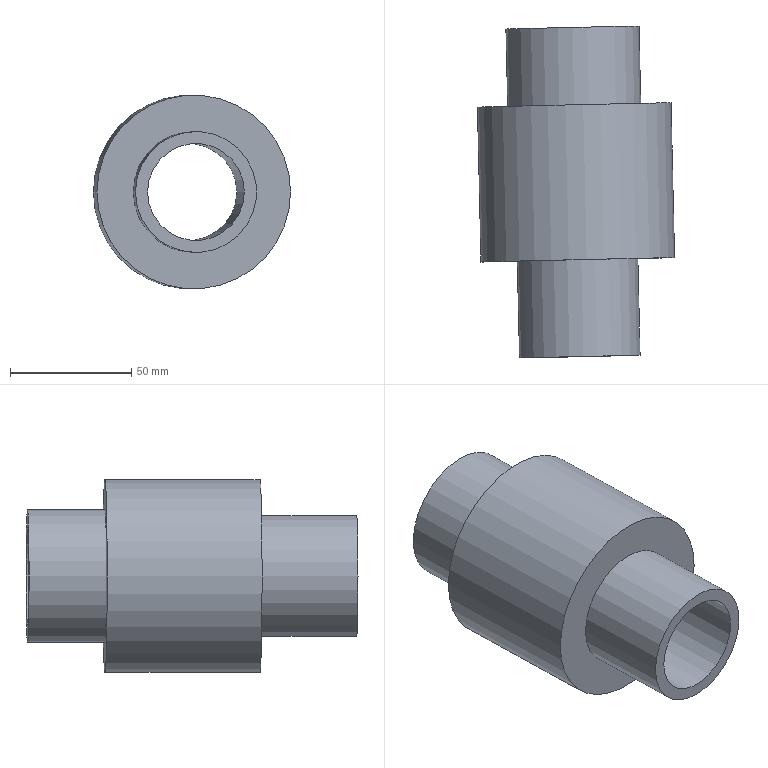Component | NX | 3 | 1 solid | 8 faces | box 81.44 x 137.16 x 80 mm | volume 305363 mm3 | plane 4 | cylinder 4 | commonest cylinder face diameters 40 x1 50 x1 80 x1 55 x1
STEP:
#1=CARTESIAN_POINT('',(0.,0.,0.));
#2=DIRECTION('',(0.,0.,1.));
#3=DIRECTION('',(1.,0.,0.));
#4=AXIS2_PLACEMENT_3D('',#1,#2,#3);
#5=CARTESIAN_POINT('',(-404.632,524.19,168.288));
#6=VERTEX_POINT('',#5);
#7=CARTESIAN_POINT('',(-384.637,524.647,168.288));
#8=DIRECTION('',(-0.02285,0.9997,0.));
#9=DIRECTION('',(-0.9997,-0.02285,0.));
#10=AXIS2_PLACEMENT_3D('',#7,#8,#9);
#11=CIRCLE('',#10,20.);
#12=CARTESIAN_POINT('',(-357.144,525.275,168.288));
#13=DIRECTION('',(0.02285,-0.9997,0.));
#14=DIRECTION('',(0.9997,0.02285,-0.));
#15=AXIS2_PLACEMENT_3D('',#12,#13,#14);
#16=PLANE('',#15);
#17=CARTESIAN_POINT('',(-47.5,-0.));
#18=CARTESIAN_POINT('',(-47.5,34.641));
#19=CARTESIAN_POINT('',(-17.5,17.321));
#20=CARTESIAN_POINT('',(12.5,-0.));
#21=CARTESIAN_POINT('',(-17.5,-17.321));
#22=CARTESIAN_POINT('',(-47.5,-34.641));
#23=CARTESIAN_POINT('',(-47.5,-0.));
#24=(BOUNDED_CURVE()B_SPLINE_CURVE(2,(#17,#18,#19,#20,#21,#22,#23),.UNSPECIFIED.,.T.,.F.)B_SPLINE_CURVE_WITH_KNOTS((1,2,2,2,2,1),(-2.094,0.,2.094,4.189,6.283,8.378),.UNSPECIFIED.)CURVE()GEOMETRIC_REPRESENTATION_ITEM()RATIONAL_B_SPLINE_CURVE((1.,0.5,1.,0.5,1.,0.5,1.))REPRESENTATION_ITEM(''));
#25=(GEOMETRIC_REPRESENTATION_CONTEXT(2)PARAMETRIC_REPRESENTATION_CONTEXT()REPRESENTATION_CONTEXT('',''));
#26=DEFINITIONAL_REPRESENTATION('',(#24),#25);
#27=PCURVE('',#16,#26);
#28=CARTESIAN_POINT('',(-381.529,388.682,168.288));
#29=DIRECTION('',(-0.02285,0.9997,0.));
#30=DIRECTION('',(-0.9997,-0.02285,0.));
#31=AXIS2_PLACEMENT_3D('',#28,#29,#30);
#32=CYLINDRICAL_SURFACE('',#31,20.);
#33=CARTESIAN_POINT('',(0.,136.));
#34=DIRECTION('',(1.,0.));
#35=VECTOR('',#34,1.);
#36=LINE('',#33,#35);
#37=(GEOMETRIC_REPRESENTATION_CONTEXT(2)PARAMETRIC_REPRESENTATION_CONTEXT()REPRESENTATION_CONTEXT('',''));
#38=DEFINITIONAL_REPRESENTATION('',(#36),#37);
#39=PCURVE('',#32,#38);
#40=SURFACE_CURVE('',#11,(#27,#39),.PCURVE_S1.);
#41=EDGE_CURVE('',#6,#6,#40,.T.);
#42=ORIENTED_EDGE('',*,*,#41,.F.);
#43=EDGE_LOOP('',(#42));
#44=FACE_BOUND('',#43,.T.);
#45=CARTESIAN_POINT('',(-412.13,524.018,168.288));
#46=VERTEX_POINT('',#45);
#47=CARTESIAN_POINT('',(-384.637,524.647,168.288));
#48=DIRECTION('',(-0.02285,0.9997,0.));
#49=DIRECTION('',(-0.9997,-0.02285,0.));
#50=AXIS2_PLACEMENT_3D('',#47,#48,#49);
#51=CIRCLE('',#50,27.5);
#52=CARTESIAN_POINT('',(-55.,-0.));
#53=CARTESIAN_POINT('',(-55.,47.631));
#54=CARTESIAN_POINT('',(-13.75,23.816));
#55=CARTESIAN_POINT('',(27.5,-0.));
#56=CARTESIAN_POINT('',(-13.75,-23.816));
#57=CARTESIAN_POINT('',(-55.,-47.631));
#58=CARTESIAN_POINT('',(-55.,-0.));
#59=(BOUNDED_CURVE()B_SPLINE_CURVE(2,(#52,#53,#54,#55,#56,#57,#58),.UNSPECIFIED.,.T.,.F.)B_SPLINE_CURVE_WITH_KNOTS((1,2,2,2,2,1),(-2.094,0.,2.094,4.189,6.283,8.378),.UNSPECIFIED.)CURVE()GEOMETRIC_REPRESENTATION_ITEM()RATIONAL_B_SPLINE_CURVE((1.,0.5,1.,0.5,1.,0.5,1.))REPRESENTATION_ITEM(''));
#60=(GEOMETRIC_REPRESENTATION_CONTEXT(2)PARAMETRIC_REPRESENTATION_CONTEXT()REPRESENTATION_CONTEXT('',''));
#61=DEFINITIONAL_REPRESENTATION('',(#59),#60);
#62=PCURVE('',#16,#61);
#63=CARTESIAN_POINT('',(-381.529,388.682,168.288));
#64=DIRECTION('',(-0.02285,0.9997,0.));
#65=DIRECTION('',(-0.9997,-0.02285,0.));
#66=AXIS2_PLACEMENT_3D('',#63,#64,#65);
#67=CYLINDRICAL_SURFACE('',#66,27.5);
#68=CARTESIAN_POINT('',(0.,136.));
#69=DIRECTION('',(1.,0.));
#70=VECTOR('',#69,1.);
#71=LINE('',#68,#70);
#72=(GEOMETRIC_REPRESENTATION_CONTEXT(2)PARAMETRIC_REPRESENTATION_CONTEXT()REPRESENTATION_CONTEXT('',''));
#73=DEFINITIONAL_REPRESENTATION('',(#71),#72);
#74=PCURVE('',#67,#73);
#75=SURFACE_CURVE('',#51,(#62,#74),.PCURVE_S1.);
#76=EDGE_CURVE('',#46,#46,#75,.T.);
#77=ORIENTED_EDGE('',*,*,#76,.T.);
#78=EDGE_LOOP('',(#77));
#79=FACE_BOUND('',#78,.T.);
#80=ADVANCED_FACE('',(#44,#79),#16,.F.);
#81=CARTESIAN_POINT('',(-401.524,388.225,168.288));
#82=VERTEX_POINT('',#81);
#83=CARTESIAN_POINT('',(-381.529,388.682,168.288));
#84=DIRECTION('',(-0.02285,0.9997,0.));
#85=DIRECTION('',(-0.9997,-0.02285,0.));
#86=AXIS2_PLACEMENT_3D('',#83,#84,#85);
#87=CIRCLE('',#86,20.);
#88=CARTESIAN_POINT('',(0.,-0.));
#89=DIRECTION('',(1.,0.));
#90=VECTOR('',#89,1.);
#91=LINE('',#88,#90);
#92=(GEOMETRIC_REPRESENTATION_CONTEXT(2)PARAMETRIC_REPRESENTATION_CONTEXT()REPRESENTATION_CONTEXT('',''));
#93=DEFINITIONAL_REPRESENTATION('',(#91),#92);
#94=PCURVE('',#32,#93);
#95=CARTESIAN_POINT('',(-361.534,389.139,168.288));
#96=DIRECTION('',(-0.02285,0.9997,0.));
#97=DIRECTION('',(-0.9997,-0.02285,0.));
#98=AXIS2_PLACEMENT_3D('',#95,#96,#97);
#99=PLANE('',#98);
#100=CARTESIAN_POINT('',(20.,-0.));
#101=DIRECTION('',(1.,-0.));
#102=AXIS2_PLACEMENT_2D('',#100,#101);
#103=CIRCLE('',#102,20.);
#104=(GEOMETRIC_REPRESENTATION_CONTEXT(2)PARAMETRIC_REPRESENTATION_CONTEXT()REPRESENTATION_CONTEXT('',''));
#105=DEFINITIONAL_REPRESENTATION('',(#103),#104);
#106=PCURVE('',#99,#105);
#107=SURFACE_CURVE('',#87,(#94,#106),.PCURVE_S1.);
#108=EDGE_CURVE('',#82,#82,#107,.T.);
#109=ORIENTED_EDGE('',*,*,#108,.T.);
#110=CARTESIAN_POINT('',(-401.524,388.225,168.288));
#111=CARTESIAN_POINT('',(-404.632,524.19,168.288));
#112=B_SPLINE_CURVE_WITH_KNOTS('',1,(#110,#111),.UNSPECIFIED.,.F.,.F.,(2,2),(-0.,136.),.PIECEWISE_BEZIER_KNOTS.);
#113=CARTESIAN_POINT('',(6.283,0.));
#114=DIRECTION('',(0.,1.));
#115=VECTOR('',#114,1.);
#116=LINE('',#113,#115);
#117=(GEOMETRIC_REPRESENTATION_CONTEXT(2)PARAMETRIC_REPRESENTATION_CONTEXT()REPRESENTATION_CONTEXT('',''));
#118=DEFINITIONAL_REPRESENTATION('',(#116),#117);
#119=PCURVE('',#32,#118);
#120=CARTESIAN_POINT('',(0.,0.));
#121=DIRECTION('',(0.,1.));
#122=VECTOR('',#121,1.);
#123=LINE('',#120,#122);
#124=(GEOMETRIC_REPRESENTATION_CONTEXT(2)PARAMETRIC_REPRESENTATION_CONTEXT()REPRESENTATION_CONTEXT('',''));
#125=DEFINITIONAL_REPRESENTATION('',(#123),#124);
#126=PCURVE('',#32,#125);
#127=SEAM_CURVE('',#112,(#119,#126),.PCURVE_S1.);
#128=EDGE_CURVE('',#82,#6,#127,.T.);
#129=ORIENTED_EDGE('',*,*,#128,.T.);
#130=ORIENTED_EDGE('',*,*,#41,.F.);
#131=ORIENTED_EDGE('',*,*,#128,.F.);
#132=EDGE_LOOP('',(#109,#129,#130,#131));
#133=FACE_BOUND('',#132,.F.);
#134=ADVANCED_FACE('',(#133),#32,.F.);
#135=CARTESIAN_POINT('',(-406.522,388.111,168.288));
#136=VERTEX_POINT('',#135);
#137=CARTESIAN_POINT('',(-381.529,388.682,168.288));
#138=DIRECTION('',(-0.02285,0.9997,0.));
#139=DIRECTION('',(-0.9997,-0.02285,0.));
#140=AXIS2_PLACEMENT_3D('',#137,#138,#139);
#141=CIRCLE('',#140,25.);
#142=CARTESIAN_POINT('',(20.,-0.));
#143=DIRECTION('',(1.,-0.));
#144=AXIS2_PLACEMENT_2D('',#142,#143);
#145=CIRCLE('',#144,25.);
#146=(GEOMETRIC_REPRESENTATION_CONTEXT(2)PARAMETRIC_REPRESENTATION_CONTEXT()REPRESENTATION_CONTEXT('',''));
#147=DEFINITIONAL_REPRESENTATION('',(#145),#146);
#148=PCURVE('',#99,#147);
#149=CARTESIAN_POINT('',(-381.529,388.682,168.288));
#150=DIRECTION('',(-0.02285,0.9997,0.));
#151=DIRECTION('',(-0.9997,-0.02285,0.));
#152=AXIS2_PLACEMENT_3D('',#149,#150,#151);
#153=CYLINDRICAL_SURFACE('',#152,25.);
#154=CARTESIAN_POINT('',(0.,0.));
#155=DIRECTION('',(1.,0.));
#156=VECTOR('',#155,1.);
#157=LINE('',#154,#156);
#158=(GEOMETRIC_REPRESENTATION_CONTEXT(2)PARAMETRIC_REPRESENTATION_CONTEXT()REPRESENTATION_CONTEXT('',''));
#159=DEFINITIONAL_REPRESENTATION('',(#157),#158);
#160=PCURVE('',#153,#159);
#161=SURFACE_CURVE('',#141,(#148,#160),.PCURVE_S1.);
#162=EDGE_CURVE('',#136,#136,#161,.T.);
#163=ORIENTED_EDGE('',*,*,#162,.F.);
#164=EDGE_LOOP('',(#163));
#165=FACE_BOUND('',#164,.T.);
#166=ORIENTED_EDGE('',*,*,#108,.T.);
#167=EDGE_LOOP('',(#166));
#168=FACE_BOUND('',#167,.T.);
#169=ADVANCED_FACE('',(#165,#168),#99,.F.);
#170=CARTESIAN_POINT('',(-407.437,428.1,168.288));
#171=VERTEX_POINT('',#170);
#172=CARTESIAN_POINT('',(-382.443,428.672,168.288));
#173=DIRECTION('',(-0.02285,0.9997,0.));
#174=DIRECTION('',(-0.9997,-0.02285,0.));
#175=AXIS2_PLACEMENT_3D('',#172,#173,#174);
#176=CIRCLE('',#175,25.);
#177=CARTESIAN_POINT('',(0.,40.));
#178=DIRECTION('',(1.,0.));
#179=VECTOR('',#178,1.);
#180=LINE('',#177,#179);
#181=(GEOMETRIC_REPRESENTATION_CONTEXT(2)PARAMETRIC_REPRESENTATION_CONTEXT()REPRESENTATION_CONTEXT('',''));
#182=DEFINITIONAL_REPRESENTATION('',(#180),#181);
#183=PCURVE('',#153,#182);
#184=CARTESIAN_POINT('',(-357.45,429.243,168.288));
#185=DIRECTION('',(-0.02285,0.9997,0.));
#186=DIRECTION('',(-0.9997,-0.02285,0.));
#187=AXIS2_PLACEMENT_3D('',#184,#185,#186);
#188=PLANE('',#187);
#189=CARTESIAN_POINT('',(25.,-0.));
#190=DIRECTION('',(1.,-0.));
#191=AXIS2_PLACEMENT_2D('',#189,#190);
#192=CIRCLE('',#191,25.);
#193=(GEOMETRIC_REPRESENTATION_CONTEXT(2)PARAMETRIC_REPRESENTATION_CONTEXT()REPRESENTATION_CONTEXT('',''));
#194=DEFINITIONAL_REPRESENTATION('',(#192),#193);
#195=PCURVE('',#188,#194);
#196=SURFACE_CURVE('',#176,(#183,#195),.PCURVE_S1.);
#197=EDGE_CURVE('',#171,#171,#196,.T.);
#198=ORIENTED_EDGE('',*,*,#197,.F.);
#199=CARTESIAN_POINT('',(-406.522,388.111,168.288));
#200=CARTESIAN_POINT('',(-407.437,428.1,168.288));
#201=B_SPLINE_CURVE_WITH_KNOTS('',1,(#199,#200),.UNSPECIFIED.,.F.,.F.,(2,2),(0.,40.),.PIECEWISE_BEZIER_KNOTS.);
#202=CARTESIAN_POINT('',(0.,0.));
#203=DIRECTION('',(0.,1.));
#204=VECTOR('',#203,1.);
#205=LINE('',#202,#204);
#206=(GEOMETRIC_REPRESENTATION_CONTEXT(2)PARAMETRIC_REPRESENTATION_CONTEXT()REPRESENTATION_CONTEXT('',''));
#207=DEFINITIONAL_REPRESENTATION('',(#205),#206);
#208=PCURVE('',#153,#207);
#209=CARTESIAN_POINT('',(6.283,0.));
#210=DIRECTION('',(0.,1.));
#211=VECTOR('',#210,1.);
#212=LINE('',#209,#211);
#213=(GEOMETRIC_REPRESENTATION_CONTEXT(2)PARAMETRIC_REPRESENTATION_CONTEXT()REPRESENTATION_CONTEXT('',''));
#214=DEFINITIONAL_REPRESENTATION('',(#212),#213);
#215=PCURVE('',#153,#214);
#216=SEAM_CURVE('',#201,(#208,#215),.PCURVE_S1.);
#217=EDGE_CURVE('',#136,#171,#216,.T.);
#218=ORIENTED_EDGE('',*,*,#217,.F.);
#219=ORIENTED_EDGE('',*,*,#162,.T.);
#220=ORIENTED_EDGE('',*,*,#217,.T.);
#221=EDGE_LOOP('',(#198,#218,#219,#220));
#222=FACE_BOUND('',#221,.T.);
#223=ADVANCED_FACE('',(#222),#153,.T.);
#224=CARTESIAN_POINT('',(-422.433,427.758,168.288));
#225=VERTEX_POINT('',#224);
#226=CARTESIAN_POINT('',(-382.443,428.672,168.288));
#227=DIRECTION('',(-0.02285,0.9997,-0.));
#228=DIRECTION('',(-0.9997,-0.02285,0.));
#229=AXIS2_PLACEMENT_3D('',#226,#227,#228);
#230=CIRCLE('',#229,40.);
#231=CARTESIAN_POINT('',(25.,-0.));
#232=DIRECTION('',(1.,0.));
#233=AXIS2_PLACEMENT_2D('',#231,#232);
#234=CIRCLE('',#233,40.);
#235=(GEOMETRIC_REPRESENTATION_CONTEXT(2)PARAMETRIC_REPRESENTATION_CONTEXT()REPRESENTATION_CONTEXT('',''));
#236=DEFINITIONAL_REPRESENTATION('',(#234),#235);
#237=PCURVE('',#188,#236);
#238=CARTESIAN_POINT('',(-381.529,388.682,168.288));
#239=DIRECTION('',(-0.02285,0.9997,0.));
#240=DIRECTION('',(-0.9997,-0.02285,0.));
#241=AXIS2_PLACEMENT_3D('',#238,#239,#240);
#242=CYLINDRICAL_SURFACE('',#241,40.);
#243=CARTESIAN_POINT('',(0.,40.));
#244=DIRECTION('',(1.,0.));
#245=VECTOR('',#244,1.);
#246=LINE('',#243,#245);
#247=(GEOMETRIC_REPRESENTATION_CONTEXT(2)PARAMETRIC_REPRESENTATION_CONTEXT()REPRESENTATION_CONTEXT('',''));
#248=DEFINITIONAL_REPRESENTATION('',(#246),#247);
#249=PCURVE('',#242,#248);
#250=SURFACE_CURVE('',#230,(#237,#249),.PCURVE_S1.);
#251=EDGE_CURVE('',#225,#225,#250,.T.);
#252=ORIENTED_EDGE('',*,*,#251,.F.);
#253=EDGE_LOOP('',(#252));
#254=FACE_BOUND('',#253,.T.);
#255=ORIENTED_EDGE('',*,*,#197,.T.);
#256=EDGE_LOOP('',(#255));
#257=FACE_BOUND('',#256,.T.);
#258=ADVANCED_FACE('',(#254,#257),#188,.F.);
#259=CARTESIAN_POINT('',(-423.895,491.741,168.288));
#260=VERTEX_POINT('',#259);
#261=CARTESIAN_POINT('',(-343.916,493.569,168.288));
#262=VERTEX_POINT('',#261);
#263=CARTESIAN_POINT('',(-383.906,492.655,168.288));
#264=DIRECTION('',(-0.02285,0.9997,-0.));
#265=DIRECTION('',(0.9997,0.02285,-0.));
#266=AXIS2_PLACEMENT_3D('',#263,#264,#265);
#267=CIRCLE('',#266,40.);
#268=CARTESIAN_POINT('',(-3.142,104.));
#269=DIRECTION('',(1.,0.));
#270=VECTOR('',#269,1.);
#271=LINE('',#268,#270);
#272=(GEOMETRIC_REPRESENTATION_CONTEXT(2)PARAMETRIC_REPRESENTATION_CONTEXT()REPRESENTATION_CONTEXT('',''));
#273=DEFINITIONAL_REPRESENTATION('',(#271),#272);
#274=PCURVE('',#242,#273);
#275=CARTESIAN_POINT('',(-343.466,493.58,168.288));
#276=DIRECTION('',(0.02285,-0.9997,0.));
#277=DIRECTION('',(0.9997,0.02285,-0.));
#278=AXIS2_PLACEMENT_3D('',#275,#276,#277);
#279=PLANE('',#278);
#280=CARTESIAN_POINT('',(-0.4505,0.));
#281=CARTESIAN_POINT('',(-0.4505,-69.282));
#282=CARTESIAN_POINT('',(-60.451,-34.641));
#283=CARTESIAN_POINT('',(-120.451,0.));
#284=CARTESIAN_POINT('',(-60.451,34.641));
#285=CARTESIAN_POINT('',(-0.4505,69.282));
#286=CARTESIAN_POINT('',(-0.4505,0.));
#287=(BOUNDED_CURVE()B_SPLINE_CURVE(2,(#280,#281,#282,#283,#284,#285,#286),.UNSPECIFIED.,.T.,.F.)B_SPLINE_CURVE_WITH_KNOTS((1,2,2,2,2,1),(-2.094,0.,2.094,4.189,6.283,8.378),.UNSPECIFIED.)CURVE()GEOMETRIC_REPRESENTATION_ITEM()RATIONAL_B_SPLINE_CURVE((1.,0.5,1.,0.5,1.,0.5,1.))REPRESENTATION_ITEM(''));
#288=(GEOMETRIC_REPRESENTATION_CONTEXT(2)PARAMETRIC_REPRESENTATION_CONTEXT()REPRESENTATION_CONTEXT('',''));
#289=DEFINITIONAL_REPRESENTATION('',(#287),#288);
#290=PCURVE('',#279,#289);
#291=SURFACE_CURVE('',#267,(#274,#290),.PCURVE_S1.);
#292=EDGE_CURVE('',#260,#262,#291,.T.);
#293=ORIENTED_EDGE('',*,*,#292,.F.);
#294=CARTESIAN_POINT('',(-422.433,427.758,168.288));
#295=CARTESIAN_POINT('',(-423.895,491.741,168.288));
#296=B_SPLINE_CURVE_WITH_KNOTS('',1,(#294,#295),.UNSPECIFIED.,.F.,.F.,(2,2),(40.,104.),.PIECEWISE_BEZIER_KNOTS.);
#297=CARTESIAN_POINT('',(0.,0.));
#298=DIRECTION('',(0.,1.));
#299=VECTOR('',#298,1.);
#300=LINE('',#297,#299);
#301=(GEOMETRIC_REPRESENTATION_CONTEXT(2)PARAMETRIC_REPRESENTATION_CONTEXT()REPRESENTATION_CONTEXT('',''));
#302=DEFINITIONAL_REPRESENTATION('',(#300),#301);
#303=PCURVE('',#242,#302);
#304=CARTESIAN_POINT('',(6.283,0.));
#305=DIRECTION('',(0.,1.));
#306=VECTOR('',#305,1.);
#307=LINE('',#304,#306);
#308=(GEOMETRIC_REPRESENTATION_CONTEXT(2)PARAMETRIC_REPRESENTATION_CONTEXT()REPRESENTATION_CONTEXT('',''));
#309=DEFINITIONAL_REPRESENTATION('',(#307),#308);
#310=PCURVE('',#242,#309);
#311=SEAM_CURVE('',#296,(#303,#310),.PCURVE_S1.);
#312=EDGE_CURVE('',#225,#260,#311,.T.);
#313=ORIENTED_EDGE('',*,*,#312,.F.);
#314=ORIENTED_EDGE('',*,*,#251,.T.);
#315=ORIENTED_EDGE('',*,*,#312,.T.);
#316=CARTESIAN_POINT('',(-383.906,492.655,168.288));
#317=DIRECTION('',(-0.02285,0.9997,-0.));
#318=DIRECTION('',(0.9997,0.02285,-0.));
#319=AXIS2_PLACEMENT_3D('',#316,#317,#318);
#320=CIRCLE('',#319,40.);
#321=CARTESIAN_POINT('',(3.142,104.));
#322=DIRECTION('',(1.,0.));
#323=VECTOR('',#322,1.);
#324=LINE('',#321,#323);
#325=(GEOMETRIC_REPRESENTATION_CONTEXT(2)PARAMETRIC_REPRESENTATION_CONTEXT()REPRESENTATION_CONTEXT('',''));
#326=DEFINITIONAL_REPRESENTATION('',(#324),#325);
#327=PCURVE('',#242,#326);
#328=CARTESIAN_POINT('',(-0.4505,0.));
#329=CARTESIAN_POINT('',(-0.4505,-69.282));
#330=CARTESIAN_POINT('',(-60.451,-34.641));
#331=CARTESIAN_POINT('',(-120.451,0.));
#332=CARTESIAN_POINT('',(-60.451,34.641));
#333=CARTESIAN_POINT('',(-0.4505,69.282));
#334=CARTESIAN_POINT('',(-0.4505,0.));
#335=(BOUNDED_CURVE()B_SPLINE_CURVE(2,(#328,#329,#330,#331,#332,#333,#334),.UNSPECIFIED.,.T.,.F.)B_SPLINE_CURVE_WITH_KNOTS((1,2,2,2,2,1),(-2.094,0.,2.094,4.189,6.283,8.378),.UNSPECIFIED.)CURVE()GEOMETRIC_REPRESENTATION_ITEM()RATIONAL_B_SPLINE_CURVE((1.,0.5,1.,0.5,1.,0.5,1.))REPRESENTATION_ITEM(''));
#336=(GEOMETRIC_REPRESENTATION_CONTEXT(2)PARAMETRIC_REPRESENTATION_CONTEXT()REPRESENTATION_CONTEXT('',''));
#337=DEFINITIONAL_REPRESENTATION('',(#335),#336);
#338=PCURVE('',#279,#337);
#339=SURFACE_CURVE('',#320,(#327,#338),.PCURVE_S1.);
#340=EDGE_CURVE('',#262,#260,#339,.T.);
#341=ORIENTED_EDGE('',*,*,#340,.F.);
#342=EDGE_LOOP('',(#293,#313,#314,#315,#341));
#343=FACE_BOUND('',#342,.T.);
#344=ADVANCED_FACE('',(#343),#242,.T.);
#345=CARTESIAN_POINT('',(-411.399,492.027,168.288));
#346=VERTEX_POINT('',#345);
#347=CARTESIAN_POINT('',(-383.906,492.655,168.288));
#348=DIRECTION('',(-0.02285,0.9997,0.));
#349=DIRECTION('',(-0.9997,-0.02285,0.));
#350=AXIS2_PLACEMENT_3D('',#347,#348,#349);
#351=CIRCLE('',#350,27.5);
#352=CARTESIAN_POINT('',(-67.951,0.));
#353=CARTESIAN_POINT('',(-67.951,47.631));
#354=CARTESIAN_POINT('',(-26.701,23.816));
#355=CARTESIAN_POINT('',(14.549,0.));
#356=CARTESIAN_POINT('',(-26.701,-23.816));
#357=CARTESIAN_POINT('',(-67.951,-47.631));
#358=CARTESIAN_POINT('',(-67.951,0.));
#359=(BOUNDED_CURVE()B_SPLINE_CURVE(2,(#352,#353,#354,#355,#356,#357,#358),.UNSPECIFIED.,.T.,.F.)B_SPLINE_CURVE_WITH_KNOTS((1,2,2,2,2,1),(-2.094,0.,2.094,4.189,6.283,8.378),.UNSPECIFIED.)CURVE()GEOMETRIC_REPRESENTATION_ITEM()RATIONAL_B_SPLINE_CURVE((1.,0.5,1.,0.5,1.,0.5,1.))REPRESENTATION_ITEM(''));
#360=(GEOMETRIC_REPRESENTATION_CONTEXT(2)PARAMETRIC_REPRESENTATION_CONTEXT()REPRESENTATION_CONTEXT('',''));
#361=DEFINITIONAL_REPRESENTATION('',(#359),#360);
#362=PCURVE('',#279,#361);
#363=CARTESIAN_POINT('',(0.,104.));
#364=DIRECTION('',(1.,0.));
#365=VECTOR('',#364,1.);
#366=LINE('',#363,#365);
#367=(GEOMETRIC_REPRESENTATION_CONTEXT(2)PARAMETRIC_REPRESENTATION_CONTEXT()REPRESENTATION_CONTEXT('',''));
#368=DEFINITIONAL_REPRESENTATION('',(#366),#367);
#369=PCURVE('',#67,#368);
#370=SURFACE_CURVE('',#351,(#362,#369),.PCURVE_S1.);
#371=EDGE_CURVE('',#346,#346,#370,.T.);
#372=ORIENTED_EDGE('',*,*,#371,.F.);
#373=EDGE_LOOP('',(#372));
#374=FACE_BOUND('',#373,.T.);
#375=ORIENTED_EDGE('',*,*,#340,.T.);
#376=ORIENTED_EDGE('',*,*,#292,.T.);
#377=EDGE_LOOP('',(#375,#376));
#378=FACE_BOUND('',#377,.T.);
#379=ADVANCED_FACE('',(#374,#378),#279,.F.);
#380=ORIENTED_EDGE('',*,*,#76,.F.);
#381=CARTESIAN_POINT('',(-411.399,492.027,168.288));
#382=CARTESIAN_POINT('',(-412.13,524.018,168.288));
#383=B_SPLINE_CURVE_WITH_KNOTS('',1,(#381,#382),.UNSPECIFIED.,.F.,.F.,(2,2),(104.,136.),.PIECEWISE_BEZIER_KNOTS.);
#384=CARTESIAN_POINT('',(0.,0.));
#385=DIRECTION('',(0.,1.));
#386=VECTOR('',#385,1.);
#387=LINE('',#384,#386);
#388=(GEOMETRIC_REPRESENTATION_CONTEXT(2)PARAMETRIC_REPRESENTATION_CONTEXT()REPRESENTATION_CONTEXT('',''));
#389=DEFINITIONAL_REPRESENTATION('',(#387),#388);
#390=PCURVE('',#67,#389);
#391=CARTESIAN_POINT('',(6.283,0.));
#392=DIRECTION('',(0.,1.));
#393=VECTOR('',#392,1.);
#394=LINE('',#391,#393);
#395=(GEOMETRIC_REPRESENTATION_CONTEXT(2)PARAMETRIC_REPRESENTATION_CONTEXT()REPRESENTATION_CONTEXT('',''));
#396=DEFINITIONAL_REPRESENTATION('',(#394),#395);
#397=PCURVE('',#67,#396);
#398=SEAM_CURVE('',#383,(#390,#397),.PCURVE_S1.);
#399=EDGE_CURVE('',#346,#46,#398,.T.);
#400=ORIENTED_EDGE('',*,*,#399,.F.);
#401=ORIENTED_EDGE('',*,*,#371,.T.);
#402=ORIENTED_EDGE('',*,*,#399,.T.);
#403=EDGE_LOOP('',(#380,#400,#401,#402));
#404=FACE_BOUND('',#403,.T.);
#405=ADVANCED_FACE('',(#404),#67,.T.);
#406=CLOSED_SHELL('',(#80,#134,#169,#223,#258,#344,#379,#405));
#407=MANIFOLD_SOLID_BREP('',#406);
#408=(LENGTH_UNIT()NAMED_UNIT(*)SI_UNIT(.MILLI.,.METRE.));
#409=UNCERTAINTY_MEASURE_WITH_UNIT(LENGTH_MEASURE(0.000005),#408,'','');
#410=(NAMED_UNIT(*)PLANE_ANGLE_UNIT()SI_UNIT($,.RADIAN.));
#411=(NAMED_UNIT(*)SI_UNIT($,.STERADIAN.)SOLID_ANGLE_UNIT());
#412=(GEOMETRIC_REPRESENTATION_CONTEXT(3)GLOBAL_UNCERTAINTY_ASSIGNED_CONTEXT((#409))GLOBAL_UNIT_ASSIGNED_CONTEXT((#408,#410,#411))REPRESENTATION_CONTEXT('',''));
#413=ADVANCED_BREP_SHAPE_REPRESENTATION('',(#4,#407),#412);